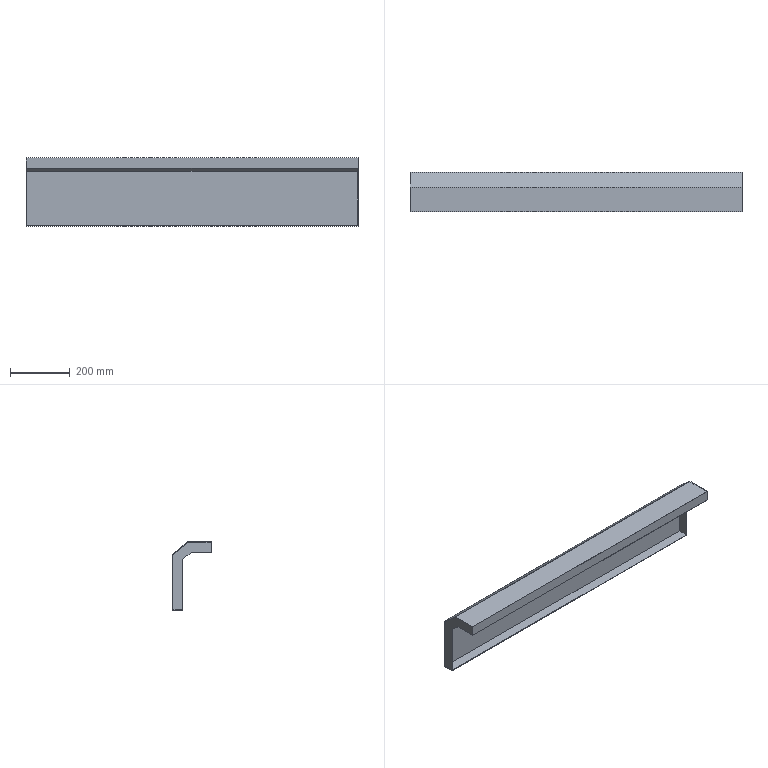Component | SolidWorks | UpperBaffle-1 | 1 solid | 18 faces | box 1110 x 132 x 228 mm | volume 921389 mm3 | plane 18
STEP:
#1=COLOUR_RGB('',0.7922,0.8196,0.9333);
#2=FILL_AREA_STYLE_COLOUR('',#1);
#3=FILL_AREA_STYLE('',(#2));
#4=SURFACE_STYLE_FILL_AREA(#3);
#5=SURFACE_SIDE_STYLE('',(#4));
#6=SURFACE_STYLE_USAGE(.BOTH.,#5);
#7=PRESENTATION_STYLE_ASSIGNMENT((#6));
#8=CARTESIAN_POINT('',(9.388,19.324,6.985));
#9=VERTEX_POINT('',#8);
#10=CARTESIAN_POINT('',(9.388,16.203,6.985));
#11=VERTEX_POINT('',#10);
#12=CARTESIAN_POINT('',(9.388,19.141,6.985));
#13=DIRECTION('',(0.,-1.,0.));
#14=VECTOR('',#13,39.37);
#15=LINE('',#12,#14);
#16=EDGE_CURVE('',#9,#11,#15,.T.);
#17=ORIENTED_EDGE('',*,*,#16,.T.);
#18=CARTESIAN_POINT('',(-34.155,16.203,6.985));
#19=VERTEX_POINT('',#18);
#20=CARTESIAN_POINT('',(9.467,16.203,6.985));
#21=DIRECTION('',(-1.,-0.,-0.));
#22=VECTOR('',#21,39.37);
#23=LINE('',#20,#22);
#24=EDGE_CURVE('',#11,#19,#23,.T.);
#25=ORIENTED_EDGE('',*,*,#24,.T.);
#26=CARTESIAN_POINT('',(-34.155,19.324,6.985));
#27=VERTEX_POINT('',#26);
#28=CARTESIAN_POINT('',(-34.155,19.141,6.985));
#29=DIRECTION('',(0.,-1.,0.));
#30=VECTOR('',#29,39.37);
#31=LINE('',#28,#30);
#32=EDGE_CURVE('',#27,#19,#31,.T.);
#33=ORIENTED_EDGE('',*,*,#32,.F.);
#34=CARTESIAN_POINT('',(9.467,19.324,6.985));
#35=DIRECTION('',(-1.,-0.,-0.));
#36=VECTOR('',#35,39.37);
#37=LINE('',#34,#36);
#38=EDGE_CURVE('',#9,#27,#37,.T.);
#39=ORIENTED_EDGE('',*,*,#38,.F.);
#40=EDGE_LOOP('',(#17,#25,#33,#39));
#41=FACE_OUTER_BOUND('',#40,.T.);
#42=CARTESIAN_POINT('',(9.467,16.125,6.985));
#43=DIRECTION('',(0.,0.,-1.));
#44=DIRECTION('',(-1.,-0.,-0.));
#45=AXIS2_PLACEMENT_3D('',#42,#43,#44);
#46=PLANE('',#45);
#47=ADVANCED_FACE('',(#41),#46,.T.);
#48=CARTESIAN_POINT('',(9.388,16.203,5.686));
#49=VERTEX_POINT('',#48);
#50=CARTESIAN_POINT('',(9.388,18.843,5.686));
#51=VERTEX_POINT('',#50);
#52=CARTESIAN_POINT('',(9.388,19.141,5.686));
#53=DIRECTION('',(-0.,1.,0.));
#54=VECTOR('',#53,39.37);
#55=LINE('',#52,#54);
#56=EDGE_CURVE('',#49,#51,#55,.T.);
#57=ORIENTED_EDGE('',*,*,#56,.F.);
#58=CARTESIAN_POINT('',(9.388,16.203,4.708));
#59=DIRECTION('',(-0.,-0.,1.));
#60=VECTOR('',#59,39.37);
#61=LINE('',#58,#60);
#62=EDGE_CURVE('',#49,#11,#61,.T.);
#63=ORIENTED_EDGE('',*,*,#62,.T.);
#64=ORIENTED_EDGE('',*,*,#16,.F.);
#65=CARTESIAN_POINT('',(9.388,21.243,5.337));
#66=VERTEX_POINT('',#65);
#67=CARTESIAN_POINT('',(9.388,20.344,6.109));
#68=DIRECTION('',(0.,-0.7586,0.6516));
#69=VECTOR('',#68,39.37);
#70=LINE('',#67,#69);
#71=EDGE_CURVE('',#66,#9,#70,.T.);
#72=ORIENTED_EDGE('',*,*,#71,.F.);
#73=CARTESIAN_POINT('',(9.388,21.243,-1.833));
#74=VERTEX_POINT('',#73);
#75=CARTESIAN_POINT('',(9.388,21.243,4.708));
#76=DIRECTION('',(-0.,0.,1.));
#77=VECTOR('',#76,39.37);
#78=LINE('',#75,#77);
#79=EDGE_CURVE('',#74,#66,#78,.T.);
#80=ORIENTED_EDGE('',*,*,#79,.F.);
#81=CARTESIAN_POINT('',(9.388,19.944,-1.833));
#82=VERTEX_POINT('',#81);
#83=CARTESIAN_POINT('',(9.388,19.141,-1.833));
#84=DIRECTION('',(-0.,1.,-0.));
#85=VECTOR('',#84,39.37);
#86=LINE('',#83,#85);
#87=EDGE_CURVE('',#82,#74,#86,.T.);
#88=ORIENTED_EDGE('',*,*,#87,.F.);
#89=CARTESIAN_POINT('',(9.388,19.944,4.741));
#90=VERTEX_POINT('',#89);
#91=CARTESIAN_POINT('',(9.388,19.944,4.708));
#92=DIRECTION('',(0.,0.,-1.));
#93=VECTOR('',#92,39.37);
#94=LINE('',#91,#93);
#95=EDGE_CURVE('',#90,#82,#94,.T.);
#96=ORIENTED_EDGE('',*,*,#95,.F.);
#97=CARTESIAN_POINT('',(9.388,19.498,5.124));
#98=DIRECTION('',(-0.,0.7586,-0.6516));
#99=VECTOR('',#98,39.37);
#100=LINE('',#97,#99);
#101=EDGE_CURVE('',#51,#90,#100,.T.);
#102=ORIENTED_EDGE('',*,*,#101,.F.);
#103=EDGE_LOOP('',(#57,#63,#64,#72,#80,#88,#96,#102));
#104=FACE_OUTER_BOUND('',#103,.T.);
#105=CARTESIAN_POINT('',(9.388,19.141,4.708));
#106=DIRECTION('',(-1.,-0.,-0.));
#107=DIRECTION('',(-0.,0.,1.));
#108=AXIS2_PLACEMENT_3D('',#105,#106,#107);
#109=PLANE('',#108);
#110=ADVANCED_FACE('',(#104),#109,.T.);
#111=CARTESIAN_POINT('',(-34.155,16.203,5.686));
#112=VERTEX_POINT('',#111);
#113=CARTESIAN_POINT('',(-34.155,16.203,4.708));
#114=DIRECTION('',(-0.,-0.,1.));
#115=VECTOR('',#114,39.37);
#116=LINE('',#113,#115);
#117=EDGE_CURVE('',#112,#19,#116,.T.);
#118=ORIENTED_EDGE('',*,*,#117,.F.);
#119=CARTESIAN_POINT('',(-34.155,18.843,5.686));
#120=VERTEX_POINT('',#119);
#121=CARTESIAN_POINT('',(-34.155,19.141,5.686));
#122=DIRECTION('',(-0.,1.,0.));
#123=VECTOR('',#122,39.37);
#124=LINE('',#121,#123);
#125=EDGE_CURVE('',#112,#120,#124,.T.);
#126=ORIENTED_EDGE('',*,*,#125,.T.);
#127=CARTESIAN_POINT('',(-34.155,19.944,4.741));
#128=VERTEX_POINT('',#127);
#129=CARTESIAN_POINT('',(-34.155,19.498,5.124));
#130=DIRECTION('',(-0.,0.7586,-0.6516));
#131=VECTOR('',#130,39.37);
#132=LINE('',#129,#131);
#133=EDGE_CURVE('',#120,#128,#132,.T.);
#134=ORIENTED_EDGE('',*,*,#133,.T.);
#135=CARTESIAN_POINT('',(-34.155,19.944,-1.833));
#136=VERTEX_POINT('',#135);
#137=CARTESIAN_POINT('',(-34.155,19.944,4.708));
#138=DIRECTION('',(0.,0.,-1.));
#139=VECTOR('',#138,39.37);
#140=LINE('',#137,#139);
#141=EDGE_CURVE('',#128,#136,#140,.T.);
#142=ORIENTED_EDGE('',*,*,#141,.T.);
#143=CARTESIAN_POINT('',(-34.155,21.243,-1.833));
#144=VERTEX_POINT('',#143);
#145=CARTESIAN_POINT('',(-34.155,19.141,-1.833));
#146=DIRECTION('',(-0.,1.,-0.));
#147=VECTOR('',#146,39.37);
#148=LINE('',#145,#147);
#149=EDGE_CURVE('',#136,#144,#148,.T.);
#150=ORIENTED_EDGE('',*,*,#149,.T.);
#151=CARTESIAN_POINT('',(-34.155,21.243,5.337));
#152=VERTEX_POINT('',#151);
#153=CARTESIAN_POINT('',(-34.155,21.243,4.708));
#154=DIRECTION('',(-0.,0.,1.));
#155=VECTOR('',#154,39.37);
#156=LINE('',#153,#155);
#157=EDGE_CURVE('',#144,#152,#156,.T.);
#158=ORIENTED_EDGE('',*,*,#157,.T.);
#159=CARTESIAN_POINT('',(-34.155,20.344,6.109));
#160=DIRECTION('',(0.,-0.7586,0.6516));
#161=VECTOR('',#160,39.37);
#162=LINE('',#159,#161);
#163=EDGE_CURVE('',#152,#27,#162,.T.);
#164=ORIENTED_EDGE('',*,*,#163,.T.);
#165=ORIENTED_EDGE('',*,*,#32,.T.);
#166=EDGE_LOOP('',(#118,#126,#134,#142,#150,#158,#164,#165));
#167=FACE_OUTER_BOUND('',#166,.T.);
#168=CARTESIAN_POINT('',(-34.155,19.141,4.708));
#169=DIRECTION('',(-1.,-0.,-0.));
#170=DIRECTION('',(-0.,0.,1.));
#171=AXIS2_PLACEMENT_3D('',#168,#169,#170);
#172=PLANE('',#171);
#173=ADVANCED_FACE('',(#167),#172,.F.);
#174=CARTESIAN_POINT('',(-34.234,16.125,5.686));
#175=VERTEX_POINT('',#174);
#176=CARTESIAN_POINT('',(9.467,16.125,5.686));
#177=VERTEX_POINT('',#176);
#178=CARTESIAN_POINT('',(-42.668,16.125,5.686));
#179=DIRECTION('',(1.,0.,0.));
#180=VECTOR('',#179,39.37);
#181=LINE('',#178,#180);
#182=EDGE_CURVE('',#175,#177,#181,.T.);
#183=ORIENTED_EDGE('',*,*,#182,.T.);
#184=CARTESIAN_POINT('',(9.467,16.125,7.064));
#185=VERTEX_POINT('',#184);
#186=CARTESIAN_POINT('',(9.467,16.125,-1.912));
#187=DIRECTION('',(0.,0.,-1.));
#188=VECTOR('',#187,39.37);
#189=LINE('',#186,#188);
#190=EDGE_CURVE('',#185,#177,#189,.T.);
#191=ORIENTED_EDGE('',*,*,#190,.F.);
#192=CARTESIAN_POINT('',(-34.234,16.125,7.064));
#193=VERTEX_POINT('',#192);
#194=CARTESIAN_POINT('',(9.467,16.125,7.064));
#195=DIRECTION('',(-1.,-0.,-0.));
#196=VECTOR('',#195,39.37);
#197=LINE('',#194,#196);
#198=EDGE_CURVE('',#185,#193,#197,.T.);
#199=ORIENTED_EDGE('',*,*,#198,.T.);
#200=CARTESIAN_POINT('',(-34.234,16.125,-1.912));
#201=DIRECTION('',(0.,0.,-1.));
#202=VECTOR('',#201,39.37);
#203=LINE('',#200,#202);
#204=EDGE_CURVE('',#193,#175,#203,.T.);
#205=ORIENTED_EDGE('',*,*,#204,.T.);
#206=EDGE_LOOP('',(#183,#191,#199,#205));
#207=FACE_OUTER_BOUND('',#206,.T.);
#208=CARTESIAN_POINT('',(9.467,16.125,-1.912));
#209=DIRECTION('',(-0.,1.,0.));
#210=DIRECTION('',(-0.,-0.,1.));
#211=AXIS2_PLACEMENT_3D('',#208,#209,#210);
#212=PLANE('',#211);
#213=ADVANCED_FACE('',(#207),#212,.F.);
#214=CARTESIAN_POINT('',(9.467,19.944,-1.912));
#215=VERTEX_POINT('',#214);
#216=CARTESIAN_POINT('',(9.467,21.322,-1.912));
#217=VERTEX_POINT('',#216);
#218=CARTESIAN_POINT('',(9.467,21.322,-1.912));
#219=DIRECTION('',(-0.,1.,-0.));
#220=VECTOR('',#219,39.37);
#221=LINE('',#218,#220);
#222=EDGE_CURVE('',#215,#217,#221,.T.);
#223=ORIENTED_EDGE('',*,*,#222,.F.);
#224=CARTESIAN_POINT('',(-34.234,19.944,-1.912));
#225=VERTEX_POINT('',#224);
#226=CARTESIAN_POINT('',(9.467,19.944,-1.912));
#227=DIRECTION('',(1.,0.,0.));
#228=VECTOR('',#227,39.37);
#229=LINE('',#226,#228);
#230=EDGE_CURVE('',#225,#215,#229,.T.);
#231=ORIENTED_EDGE('',*,*,#230,.F.);
#232=CARTESIAN_POINT('',(-34.234,21.322,-1.912));
#233=VERTEX_POINT('',#232);
#234=CARTESIAN_POINT('',(-34.234,21.322,-1.912));
#235=DIRECTION('',(-0.,1.,-0.));
#236=VECTOR('',#235,39.37);
#237=LINE('',#234,#236);
#238=EDGE_CURVE('',#225,#233,#237,.T.);
#239=ORIENTED_EDGE('',*,*,#238,.T.);
#240=CARTESIAN_POINT('',(9.467,21.322,-1.912));
#241=DIRECTION('',(-1.,-0.,-0.));
#242=VECTOR('',#241,39.37);
#243=LINE('',#240,#242);
#244=EDGE_CURVE('',#217,#233,#243,.T.);
#245=ORIENTED_EDGE('',*,*,#244,.F.);
#246=EDGE_LOOP('',(#223,#231,#239,#245));
#247=FACE_OUTER_BOUND('',#246,.T.);
#248=CARTESIAN_POINT('',(9.467,21.322,-1.912));
#249=DIRECTION('',(-0.,0.,1.));
#250=DIRECTION('',(1.,0.,0.));
#251=AXIS2_PLACEMENT_3D('',#248,#249,#250);
#252=PLANE('',#251);
#253=ADVANCED_FACE('',(#247),#252,.F.);
#254=CARTESIAN_POINT('',(-34.234,21.322,5.373));
#255=VERTEX_POINT('',#254);
#256=CARTESIAN_POINT('',(-34.234,21.322,5.373));
#257=DIRECTION('',(-0.,0.,1.));
#258=VECTOR('',#257,39.37);
#259=LINE('',#256,#258);
#260=EDGE_CURVE('',#233,#255,#259,.T.);
#261=ORIENTED_EDGE('',*,*,#260,.T.);
#262=CARTESIAN_POINT('',(9.467,21.322,5.373));
#263=VERTEX_POINT('',#262);
#264=CARTESIAN_POINT('',(9.467,21.322,5.373));
#265=DIRECTION('',(-1.,-0.,-0.));
#266=VECTOR('',#265,39.37);
#267=LINE('',#264,#266);
#268=EDGE_CURVE('',#263,#255,#267,.T.);
#269=ORIENTED_EDGE('',*,*,#268,.F.);
#270=CARTESIAN_POINT('',(9.467,21.322,5.373));
#271=DIRECTION('',(-0.,0.,1.));
#272=VECTOR('',#271,39.37);
#273=LINE('',#270,#272);
#274=EDGE_CURVE('',#217,#263,#273,.T.);
#275=ORIENTED_EDGE('',*,*,#274,.F.);
#276=ORIENTED_EDGE('',*,*,#244,.T.);
#277=EDGE_LOOP('',(#261,#269,#275,#276));
#278=FACE_OUTER_BOUND('',#277,.T.);
#279=CARTESIAN_POINT('',(9.467,21.322,5.373));
#280=DIRECTION('',(0.,-1.,0.));
#281=DIRECTION('',(-1.,-0.,-0.));
#282=AXIS2_PLACEMENT_3D('',#279,#280,#281);
#283=PLANE('',#282);
#284=ADVANCED_FACE('',(#278),#283,.F.);
#285=CARTESIAN_POINT('',(-34.234,19.353,7.064));
#286=VERTEX_POINT('',#285);
#287=CARTESIAN_POINT('',(-34.234,19.353,7.064));
#288=DIRECTION('',(0.,-0.7586,0.6516));
#289=VECTOR('',#288,39.37);
#290=LINE('',#287,#289);
#291=EDGE_CURVE('',#255,#286,#290,.T.);
#292=ORIENTED_EDGE('',*,*,#291,.T.);
#293=CARTESIAN_POINT('',(9.467,19.353,7.064));
#294=VERTEX_POINT('',#293);
#295=CARTESIAN_POINT('',(9.467,19.353,7.064));
#296=DIRECTION('',(-1.,-0.,-0.));
#297=VECTOR('',#296,39.37);
#298=LINE('',#295,#297);
#299=EDGE_CURVE('',#294,#286,#298,.T.);
#300=ORIENTED_EDGE('',*,*,#299,.F.);
#301=CARTESIAN_POINT('',(9.467,19.353,7.064));
#302=DIRECTION('',(0.,-0.7586,0.6516));
#303=VECTOR('',#302,39.37);
#304=LINE('',#301,#303);
#305=EDGE_CURVE('',#263,#294,#304,.T.);
#306=ORIENTED_EDGE('',*,*,#305,.F.);
#307=ORIENTED_EDGE('',*,*,#268,.T.);
#308=EDGE_LOOP('',(#292,#300,#306,#307));
#309=FACE_OUTER_BOUND('',#308,.T.);
#310=CARTESIAN_POINT('',(9.467,19.353,7.064));
#311=DIRECTION('',(0.,-0.6516,-0.7586));
#312=DIRECTION('',(-0.,0.7586,-0.6516));
#313=AXIS2_PLACEMENT_3D('',#310,#311,#312);
#314=PLANE('',#313);
#315=ADVANCED_FACE('',(#309),#314,.F.);
#316=ORIENTED_EDGE('',*,*,#198,.F.);
#317=CARTESIAN_POINT('',(9.467,16.125,7.064));
#318=DIRECTION('',(0.,-1.,0.));
#319=VECTOR('',#318,39.37);
#320=LINE('',#317,#319);
#321=EDGE_CURVE('',#294,#185,#320,.T.);
#322=ORIENTED_EDGE('',*,*,#321,.F.);
#323=ORIENTED_EDGE('',*,*,#299,.T.);
#324=CARTESIAN_POINT('',(-34.234,16.125,7.064));
#325=DIRECTION('',(0.,-1.,0.));
#326=VECTOR('',#325,39.37);
#327=LINE('',#324,#326);
#328=EDGE_CURVE('',#286,#193,#327,.T.);
#329=ORIENTED_EDGE('',*,*,#328,.T.);
#330=EDGE_LOOP('',(#316,#322,#323,#329));
#331=FACE_OUTER_BOUND('',#330,.T.);
#332=CARTESIAN_POINT('',(9.467,16.125,7.064));
#333=DIRECTION('',(0.,0.,-1.));
#334=DIRECTION('',(-1.,-0.,-0.));
#335=AXIS2_PLACEMENT_3D('',#332,#333,#334);
#336=PLANE('',#335);
#337=ADVANCED_FACE('',(#331),#336,.F.);
#338=ORIENTED_EDGE('',*,*,#190,.T.);
#339=CARTESIAN_POINT('',(9.467,18.843,5.686));
#340=VERTEX_POINT('',#339);
#341=CARTESIAN_POINT('',(9.467,18.843,5.686));
#342=DIRECTION('',(0.,-1.,-0.));
#343=VECTOR('',#342,39.37);
#344=LINE('',#341,#343);
#345=EDGE_CURVE('',#340,#177,#344,.T.);
#346=ORIENTED_EDGE('',*,*,#345,.F.);
#347=CARTESIAN_POINT('',(9.467,19.944,4.741));
#348=VERTEX_POINT('',#347);
#349=CARTESIAN_POINT('',(9.467,19.944,4.741));
#350=DIRECTION('',(0.,-0.7586,0.6516));
#351=VECTOR('',#350,39.37);
#352=LINE('',#349,#351);
#353=EDGE_CURVE('',#348,#340,#352,.T.);
#354=ORIENTED_EDGE('',*,*,#353,.F.);
#355=CARTESIAN_POINT('',(9.467,19.944,-1.833));
#356=DIRECTION('',(0.,0.,-1.));
#357=VECTOR('',#356,39.37);
#358=LINE('',#355,#357);
#359=EDGE_CURVE('',#348,#215,#358,.T.);
#360=ORIENTED_EDGE('',*,*,#359,.T.);
#361=ORIENTED_EDGE('',*,*,#222,.T.);
#362=ORIENTED_EDGE('',*,*,#274,.T.);
#363=ORIENTED_EDGE('',*,*,#305,.T.);
#364=ORIENTED_EDGE('',*,*,#321,.T.);
#365=EDGE_LOOP('',(#338,#346,#354,#360,#361,#362,#363,#364));
#366=FACE_OUTER_BOUND('',#365,.T.);
#367=CARTESIAN_POINT('',(9.467,19.141,4.708));
#368=DIRECTION('',(-1.,-0.,-0.));
#369=DIRECTION('',(-0.,0.,1.));
#370=AXIS2_PLACEMENT_3D('',#367,#368,#369);
#371=PLANE('',#370);
#372=ADVANCED_FACE('',(#366),#371,.F.);
#373=ORIENTED_EDGE('',*,*,#204,.F.);
#374=ORIENTED_EDGE('',*,*,#328,.F.);
#375=ORIENTED_EDGE('',*,*,#291,.F.);
#376=ORIENTED_EDGE('',*,*,#260,.F.);
#377=ORIENTED_EDGE('',*,*,#238,.F.);
#378=CARTESIAN_POINT('',(-34.234,19.944,4.741));
#379=VERTEX_POINT('',#378);
#380=CARTESIAN_POINT('',(-34.234,19.944,-1.833));
#381=DIRECTION('',(0.,0.,-1.));
#382=VECTOR('',#381,39.37);
#383=LINE('',#380,#382);
#384=EDGE_CURVE('',#379,#225,#383,.T.);
#385=ORIENTED_EDGE('',*,*,#384,.F.);
#386=CARTESIAN_POINT('',(-34.234,18.843,5.686));
#387=VERTEX_POINT('',#386);
#388=CARTESIAN_POINT('',(-34.234,19.944,4.741));
#389=DIRECTION('',(0.,-0.7586,0.6516));
#390=VECTOR('',#389,39.37);
#391=LINE('',#388,#390);
#392=EDGE_CURVE('',#379,#387,#391,.T.);
#393=ORIENTED_EDGE('',*,*,#392,.T.);
#394=CARTESIAN_POINT('',(-34.234,18.843,5.686));
#395=DIRECTION('',(0.,-1.,-0.));
#396=VECTOR('',#395,39.37);
#397=LINE('',#394,#396);
#398=EDGE_CURVE('',#387,#175,#397,.T.);
#399=ORIENTED_EDGE('',*,*,#398,.T.);
#400=EDGE_LOOP('',(#373,#374,#375,#376,#377,#385,#393,#399));
#401=FACE_OUTER_BOUND('',#400,.T.);
#402=CARTESIAN_POINT('',(-34.234,19.141,4.708));
#403=DIRECTION('',(-1.,-0.,-0.));
#404=DIRECTION('',(-0.,0.,1.));
#405=AXIS2_PLACEMENT_3D('',#402,#403,#404);
#406=PLANE('',#405);
#407=ADVANCED_FACE('',(#401),#406,.T.);
#408=ORIENTED_EDGE('',*,*,#230,.T.);
#409=ORIENTED_EDGE('',*,*,#359,.F.);
#410=CARTESIAN_POINT('',(-42.668,19.944,4.741));
#411=DIRECTION('',(1.,0.,0.));
#412=VECTOR('',#411,39.37);
#413=LINE('',#410,#412);
#414=EDGE_CURVE('',#90,#348,#413,.T.);
#415=ORIENTED_EDGE('',*,*,#414,.F.);
#416=ORIENTED_EDGE('',*,*,#95,.T.);
#417=CARTESIAN_POINT('',(9.467,19.944,-1.833));
#418=DIRECTION('',(1.,0.,0.));
#419=VECTOR('',#418,39.37);
#420=LINE('',#417,#419);
#421=EDGE_CURVE('',#136,#82,#420,.T.);
#422=ORIENTED_EDGE('',*,*,#421,.F.);
#423=ORIENTED_EDGE('',*,*,#141,.F.);
#424=CARTESIAN_POINT('',(-42.668,19.944,4.741));
#425=DIRECTION('',(1.,0.,0.));
#426=VECTOR('',#425,39.37);
#427=LINE('',#424,#426);
#428=EDGE_CURVE('',#379,#128,#427,.T.);
#429=ORIENTED_EDGE('',*,*,#428,.F.);
#430=ORIENTED_EDGE('',*,*,#384,.T.);
#431=EDGE_LOOP('',(#408,#409,#415,#416,#422,#423,#429,#430));
#432=FACE_OUTER_BOUND('',#431,.T.);
#433=CARTESIAN_POINT('',(9.467,19.944,-1.833));
#434=DIRECTION('',(-0.,1.,-0.));
#435=DIRECTION('',(1.,0.,0.));
#436=AXIS2_PLACEMENT_3D('',#433,#434,#435);
#437=PLANE('',#436);
#438=ADVANCED_FACE('',(#432),#437,.F.);
#439=ORIENTED_EDGE('',*,*,#421,.T.);
#440=ORIENTED_EDGE('',*,*,#87,.T.);
#441=CARTESIAN_POINT('',(9.467,21.243,-1.833));
#442=DIRECTION('',(-1.,-0.,-0.));
#443=VECTOR('',#442,39.37);
#444=LINE('',#441,#443);
#445=EDGE_CURVE('',#74,#144,#444,.T.);
#446=ORIENTED_EDGE('',*,*,#445,.T.);
#447=ORIENTED_EDGE('',*,*,#149,.F.);
#448=EDGE_LOOP('',(#439,#440,#446,#447));
#449=FACE_OUTER_BOUND('',#448,.T.);
#450=CARTESIAN_POINT('',(9.467,21.322,-1.833));
#451=DIRECTION('',(-0.,0.,1.));
#452=DIRECTION('',(1.,0.,0.));
#453=AXIS2_PLACEMENT_3D('',#450,#451,#452);
#454=PLANE('',#453);
#455=ADVANCED_FACE('',(#449),#454,.T.);
#456=ORIENTED_EDGE('',*,*,#157,.F.);
#457=ORIENTED_EDGE('',*,*,#445,.F.);
#458=ORIENTED_EDGE('',*,*,#79,.T.);
#459=CARTESIAN_POINT('',(9.467,21.243,5.337));
#460=DIRECTION('',(-1.,-0.,-0.));
#461=VECTOR('',#460,39.37);
#462=LINE('',#459,#461);
#463=EDGE_CURVE('',#66,#152,#462,.T.);
#464=ORIENTED_EDGE('',*,*,#463,.T.);
#465=EDGE_LOOP('',(#456,#457,#458,#464));
#466=FACE_OUTER_BOUND('',#465,.T.);
#467=CARTESIAN_POINT('',(9.467,21.243,5.373));
#468=DIRECTION('',(0.,-1.,0.));
#469=DIRECTION('',(-1.,-0.,-0.));
#470=AXIS2_PLACEMENT_3D('',#467,#468,#469);
#471=PLANE('',#470);
#472=ADVANCED_FACE('',(#466),#471,.T.);
#473=ORIENTED_EDGE('',*,*,#163,.F.);
#474=ORIENTED_EDGE('',*,*,#463,.F.);
#475=ORIENTED_EDGE('',*,*,#71,.T.);
#476=ORIENTED_EDGE('',*,*,#38,.T.);
#477=EDGE_LOOP('',(#473,#474,#475,#476));
#478=FACE_OUTER_BOUND('',#477,.T.);
#479=CARTESIAN_POINT('',(9.467,19.302,7.004));
#480=DIRECTION('',(0.,-0.6516,-0.7586));
#481=DIRECTION('',(-0.,0.7586,-0.6516));
#482=AXIS2_PLACEMENT_3D('',#479,#480,#481);
#483=PLANE('',#482);
#484=ADVANCED_FACE('',(#478),#483,.T.);
#485=ORIENTED_EDGE('',*,*,#182,.F.);
#486=ORIENTED_EDGE('',*,*,#398,.F.);
#487=CARTESIAN_POINT('',(-42.668,18.843,5.686));
#488=DIRECTION('',(1.,0.,0.));
#489=VECTOR('',#488,39.37);
#490=LINE('',#487,#489);
#491=EDGE_CURVE('',#387,#120,#490,.T.);
#492=ORIENTED_EDGE('',*,*,#491,.T.);
#493=ORIENTED_EDGE('',*,*,#125,.F.);
#494=CARTESIAN_POINT('',(9.467,16.203,5.686));
#495=DIRECTION('',(1.,0.,0.));
#496=VECTOR('',#495,39.37);
#497=LINE('',#494,#496);
#498=EDGE_CURVE('',#112,#49,#497,.T.);
#499=ORIENTED_EDGE('',*,*,#498,.T.);
#500=ORIENTED_EDGE('',*,*,#56,.T.);
#501=CARTESIAN_POINT('',(-42.668,18.843,5.686));
#502=DIRECTION('',(1.,0.,0.));
#503=VECTOR('',#502,39.37);
#504=LINE('',#501,#503);
#505=EDGE_CURVE('',#51,#340,#504,.T.);
#506=ORIENTED_EDGE('',*,*,#505,.T.);
#507=ORIENTED_EDGE('',*,*,#345,.T.);
#508=EDGE_LOOP('',(#485,#486,#492,#493,#499,#500,#506,#507));
#509=FACE_OUTER_BOUND('',#508,.T.);
#510=CARTESIAN_POINT('',(-42.668,18.843,5.686));
#511=DIRECTION('',(-0.,-0.,1.));
#512=DIRECTION('',(0.,-1.,-0.));
#513=AXIS2_PLACEMENT_3D('',#510,#511,#512);
#514=PLANE('',#513);
#515=ADVANCED_FACE('',(#509),#514,.F.);
#516=ORIENTED_EDGE('',*,*,#491,.F.);
#517=ORIENTED_EDGE('',*,*,#392,.F.);
#518=ORIENTED_EDGE('',*,*,#428,.T.);
#519=ORIENTED_EDGE('',*,*,#133,.F.);
#520=EDGE_LOOP('',(#516,#517,#518,#519));
#521=FACE_OUTER_BOUND('',#520,.T.);
#522=CARTESIAN_POINT('',(-42.668,19.944,4.741));
#523=DIRECTION('',(-0.,0.6516,0.7586));
#524=DIRECTION('',(0.,-0.7586,0.6516));
#525=AXIS2_PLACEMENT_3D('',#522,#523,#524);
#526=PLANE('',#525);
#527=ADVANCED_FACE('',(#521),#526,.F.);
#528=ORIENTED_EDGE('',*,*,#101,.T.);
#529=ORIENTED_EDGE('',*,*,#414,.T.);
#530=ORIENTED_EDGE('',*,*,#353,.T.);
#531=ORIENTED_EDGE('',*,*,#505,.F.);
#532=EDGE_LOOP('',(#528,#529,#530,#531));
#533=FACE_OUTER_BOUND('',#532,.T.);
#534=CARTESIAN_POINT('',(-42.668,19.944,4.741));
#535=DIRECTION('',(-0.,0.6516,0.7586));
#536=DIRECTION('',(0.,-0.7586,0.6516));
#537=AXIS2_PLACEMENT_3D('',#534,#535,#536);
#538=PLANE('',#537);
#539=ADVANCED_FACE('',(#533),#538,.F.);
#540=ORIENTED_EDGE('',*,*,#62,.F.);
#541=ORIENTED_EDGE('',*,*,#498,.F.);
#542=ORIENTED_EDGE('',*,*,#117,.T.);
#543=ORIENTED_EDGE('',*,*,#24,.F.);
#544=EDGE_LOOP('',(#540,#541,#542,#543));
#545=FACE_OUTER_BOUND('',#544,.T.);
#546=CARTESIAN_POINT('',(-34.234,16.203,4.708));
#547=DIRECTION('',(0.,-1.,-0.));
#548=DIRECTION('',(0.,0.,-1.));
#549=AXIS2_PLACEMENT_3D('',#546,#547,#548);
#550=PLANE('',#549);
#551=ADVANCED_FACE('',(#545),#550,.F.);
#552=CLOSED_SHELL('',(#47,#110,#173,#213,#253,#284,#315,#337,#372,#407,#438,#455,#472,#484,#515,#527,#539,#551));
#553=MANIFOLD_SOLID_BREP('',#552);
#554=STYLED_ITEM('',(#7),#553);
#555=PRESENTATION_LAYER_ASSIGNMENT('','',(#554));
#556=(LENGTH_UNIT()NAMED_UNIT(*)SI_UNIT($,.METRE.));
#557=LENGTH_MEASURE_WITH_UNIT(LENGTH_MEASURE(0.0254),#556);
#558=DIMENSIONAL_EXPONENTS(1.,0.,0.,0.,0.,0.,0.);
#559=(CONVERSION_BASED_UNIT('',#557)LENGTH_UNIT()NAMED_UNIT(#558));
#560=UNCERTAINTY_MEASURE_WITH_UNIT(LENGTH_MEASURE(0.00001),#559,'','');
#561=(NAMED_UNIT(*)PLANE_ANGLE_UNIT()SI_UNIT($,.RADIAN.));
#562=(NAMED_UNIT(*)SI_UNIT($,.STERADIAN.)SOLID_ANGLE_UNIT());
#563=(GEOMETRIC_REPRESENTATION_CONTEXT(3)GLOBAL_UNCERTAINTY_ASSIGNED_CONTEXT((#560))GLOBAL_UNIT_ASSIGNED_CONTEXT((#559,#561,#562))REPRESENTATION_CONTEXT('',''));
#564=MECHANICAL_DESIGN_GEOMETRIC_PRESENTATION_REPRESENTATION('',(#554),#563);
#565=CARTESIAN_POINT('',(0.,0.,0.));
#566=DIRECTION('',(0.,0.,1.));
#567=DIRECTION('',(1.,0.,0.));
#568=AXIS2_PLACEMENT_3D('',#565,#566,#567);
#569=(LENGTH_UNIT()NAMED_UNIT(*)SI_UNIT($,.METRE.));
#570=LENGTH_MEASURE_WITH_UNIT(LENGTH_MEASURE(0.0254),#569);
#571=DIMENSIONAL_EXPONENTS(1.,0.,0.,0.,0.,0.,0.);
#572=(CONVERSION_BASED_UNIT('',#570)LENGTH_UNIT()NAMED_UNIT(#571));
#573=UNCERTAINTY_MEASURE_WITH_UNIT(LENGTH_MEASURE(0.00001),#572,'','');
#574=(NAMED_UNIT(*)PLANE_ANGLE_UNIT()SI_UNIT($,.RADIAN.));
#575=(NAMED_UNIT(*)SI_UNIT($,.STERADIAN.)SOLID_ANGLE_UNIT());
#576=(GEOMETRIC_REPRESENTATION_CONTEXT(3)GLOBAL_UNCERTAINTY_ASSIGNED_CONTEXT((#573))GLOBAL_UNIT_ASSIGNED_CONTEXT((#572,#574,#575))REPRESENTATION_CONTEXT('',''));
#577=ADVANCED_BREP_SHAPE_REPRESENTATION('',(#553,#568),#576);